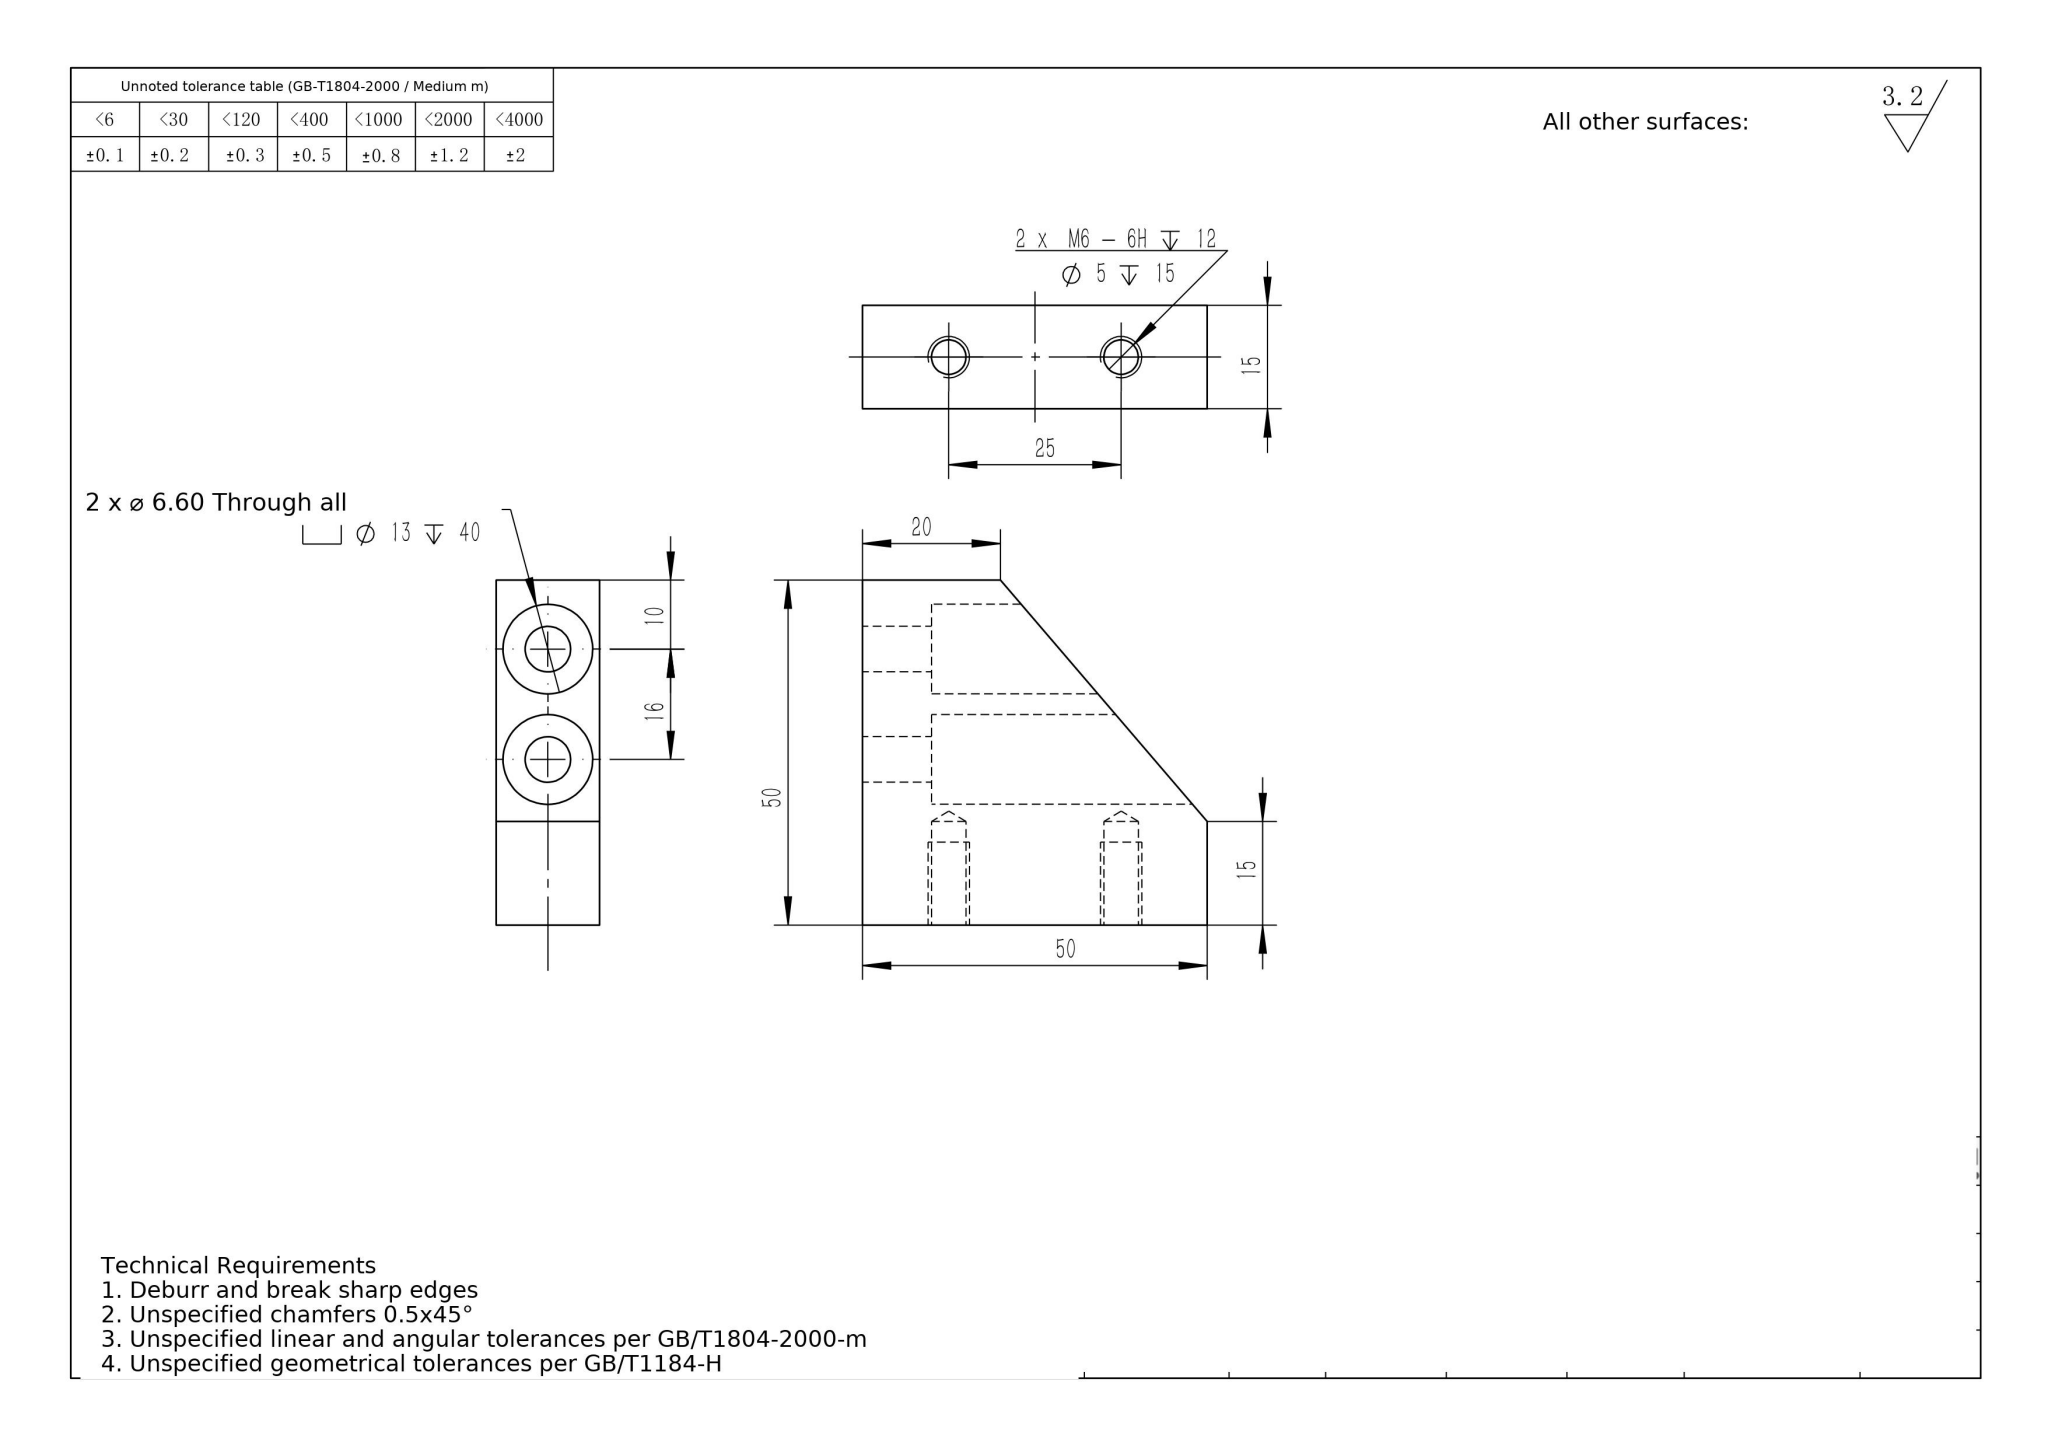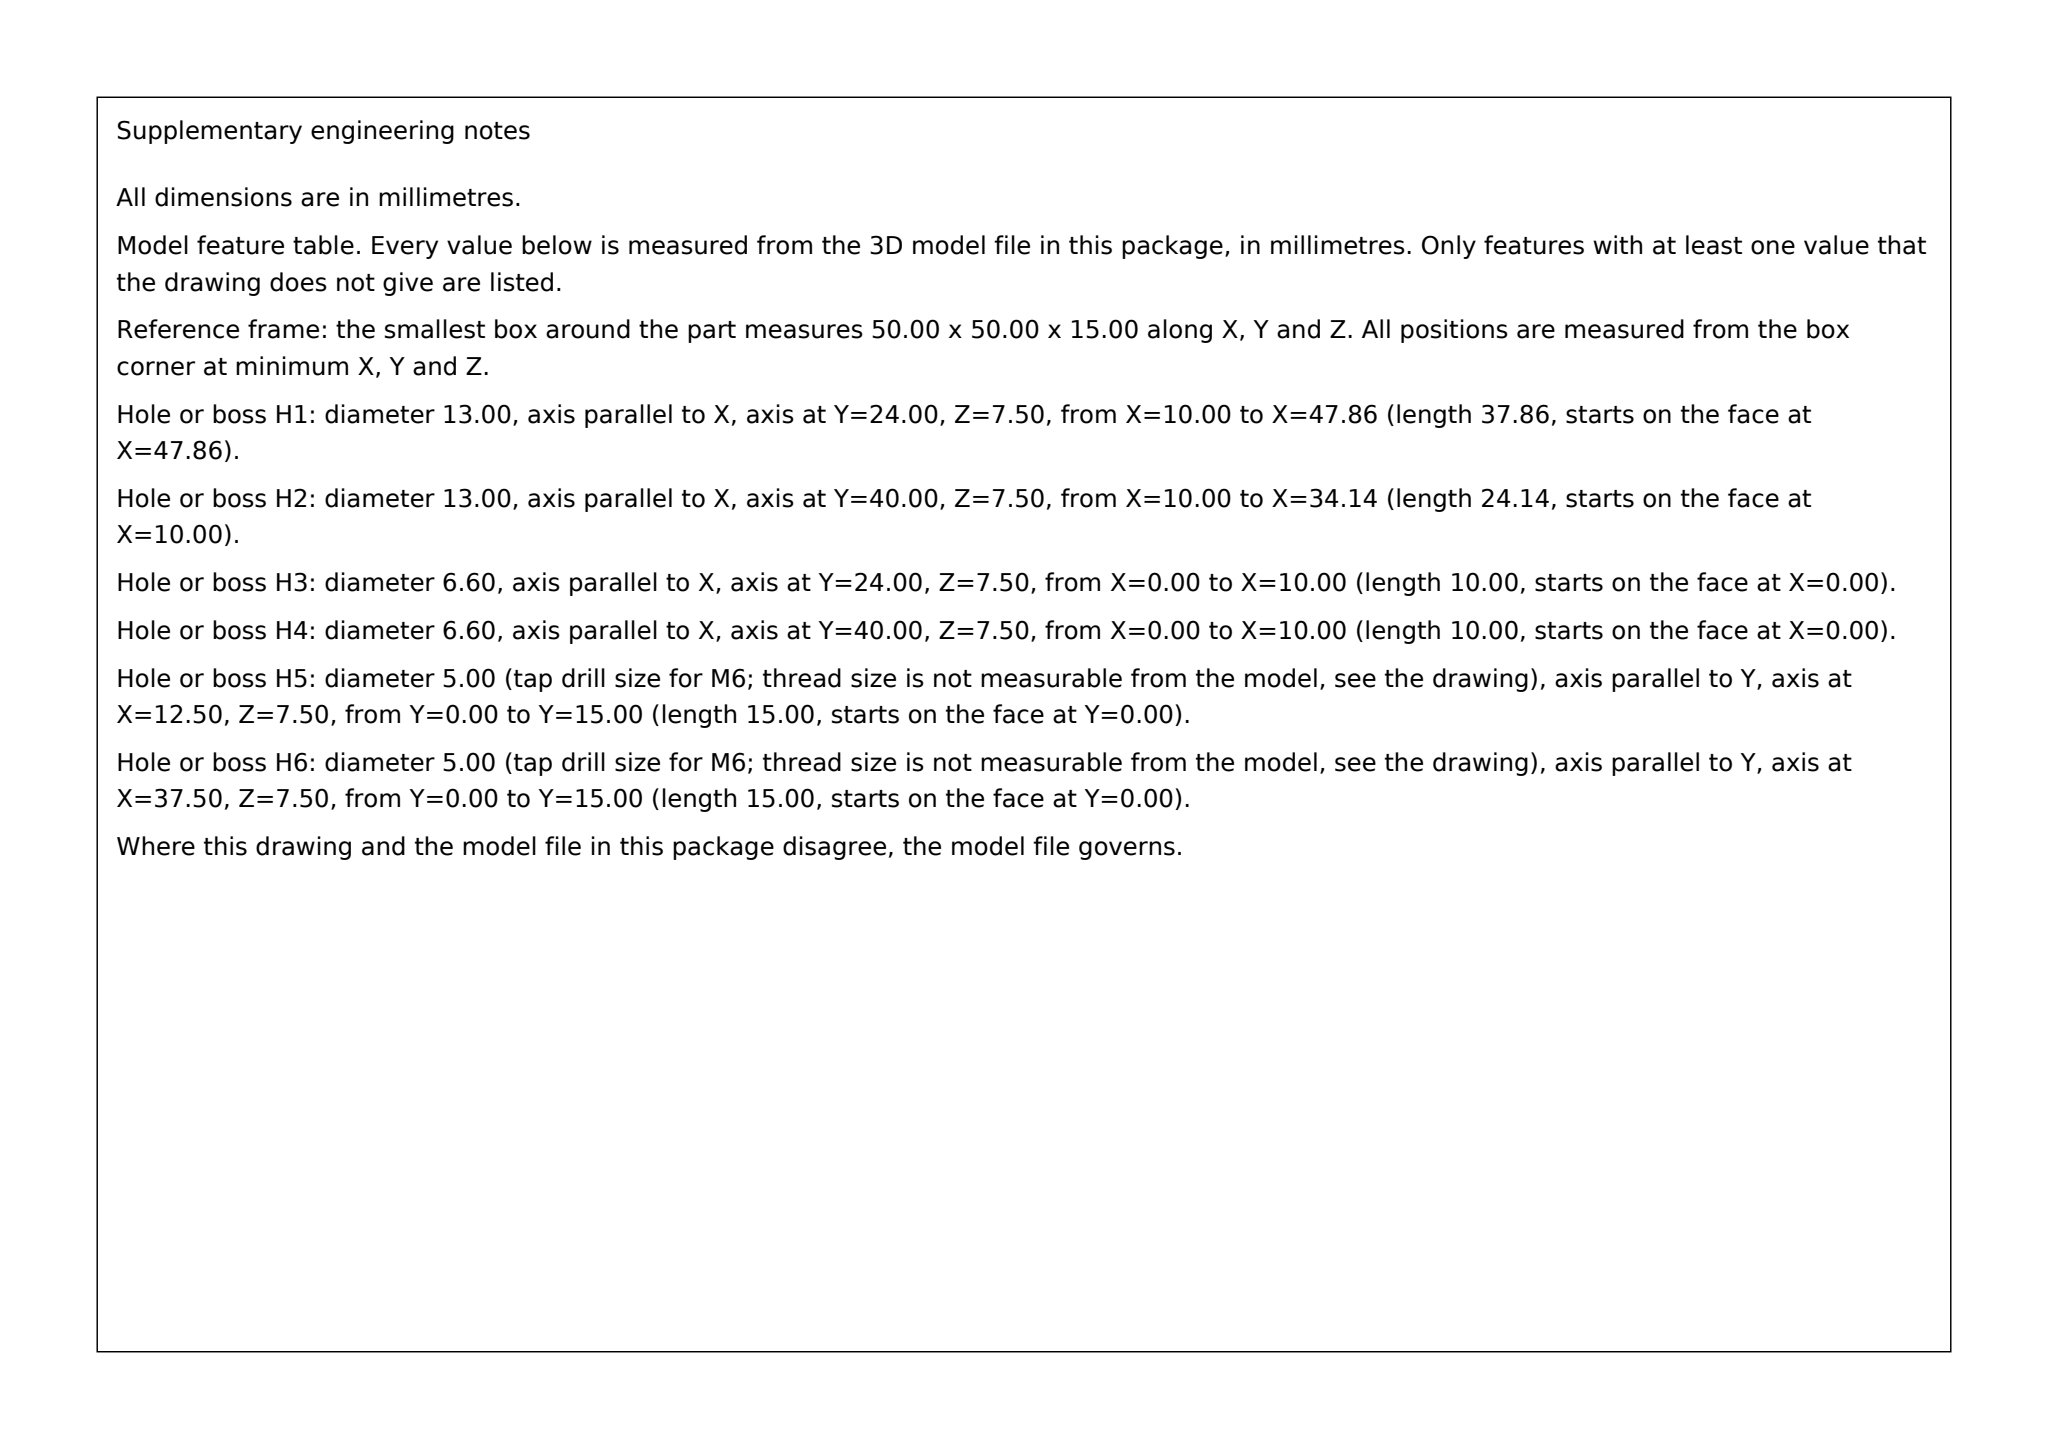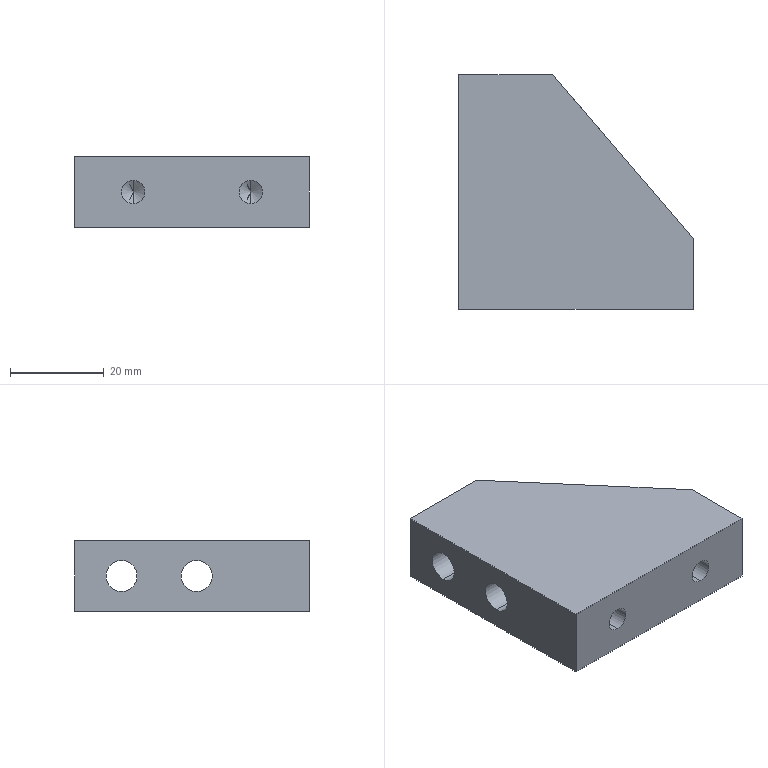Part | SolidWorks | mm | 1 solid | 25 faces | box 50 x 50 x 15 mm | volume 21582 mm3 | cylinder 12 | plane 9 | cone 4 | commonest cylinder face diameters 6.6 x4 13 x4 5 x4
build123d program:
from build123d import *

# Parameters (mm, degrees)
BOSS_EXTRUDE1_DEPTH                                  = 7.5
M6_TAPPED_HOLE1_D                                    = 5
M6_TAPPED_HOLE1_DEPTH                                = 15
M6_TAPPED_HOLE1_TIP                                  = 1.502
M6_HEX_HEAD_BOLT_CYLINDRICAL_COUNTERSUNK_D           = 6.6
M6_HEX_HEAD_BOLT_CYLINDRICAL_COUNTERSUNK_CBORE_D     = 13
M6_HEX_HEAD_BOLT_CYLINDRICAL_COUNTERSUNK_CBORE_DEPTH = 40


with BuildPart() as part:
    # Sketch1 → Boss-Extrude1 (new, symmetric)
    with BuildSketch(Plane.XY):
        Polygon((0, 50), (0, 0), (50, 0), (50, 15), (20, 50), align=None)
    extrude(amount=BOSS_EXTRUDE1_DEPTH, both=True)

    # M6 Tapped Hole1
    with Locations(Plane(origin=(0, 0, 0), x_dir=(-1, 0, 0), z_dir=(0, -1, 0))):
        with Locations((-12.5, 0), (-37.5, 0)):
            Hole(M6_TAPPED_HOLE1_D / 2, depth=M6_TAPPED_HOLE1_DEPTH)
            with Locations((0, 0, -(M6_TAPPED_HOLE1_DEPTH + M6_TAPPED_HOLE1_TIP / 2))):  # 118° drill point
                Cone(0, M6_TAPPED_HOLE1_D / 2, M6_TAPPED_HOLE1_TIP, mode=Mode.SUBTRACT)

    # M6 Hex Head Bolt Cylindrical Countersunk (through all)
    with Locations(Plane(origin=(50, 0, 0), x_dir=(0, 0, -1), z_dir=(1, 0, 0))):
        with Locations((0, 24), (0, 40)):
            CounterBoreHole(M6_HEX_HEAD_BOLT_CYLINDRICAL_COUNTERSUNK_D / 2, M6_HEX_HEAD_BOLT_CYLINDRICAL_COUNTERSUNK_CBORE_D / 2, M6_HEX_HEAD_BOLT_CYLINDRICAL_COUNTERSUNK_CBORE_DEPTH)


solid = part.part